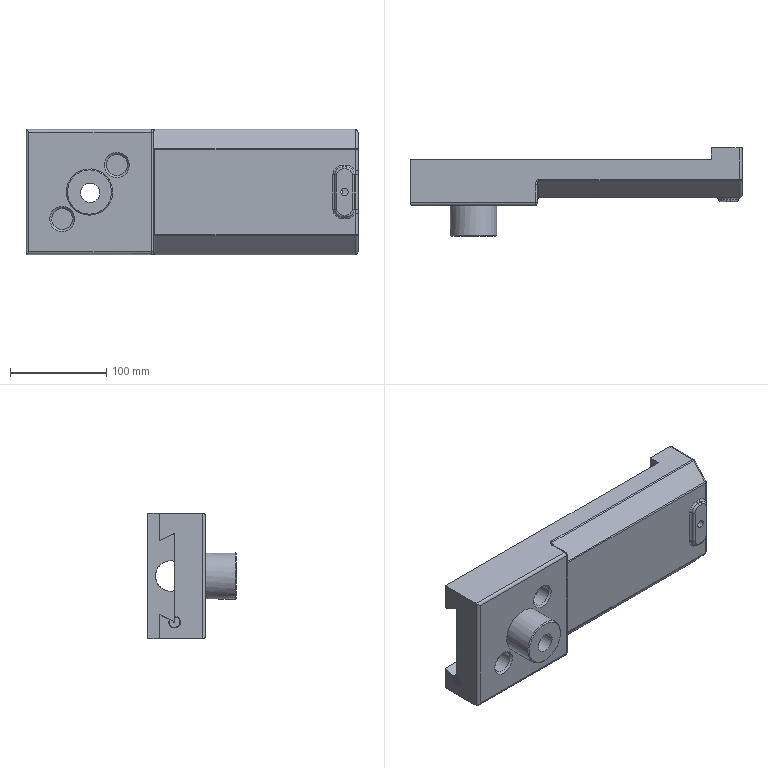Component | NX | TOOL_HOLDER_DOVETAIL_BASE | 1 solid | 175 faces | volume 1158750 mm3 | cylinder 79 | spline 50 | plane 33 | torus 10 | cone 3 | commonest cylinder face diameters 11 x21 12 x20 4 x18 6 x10 8 x4 22 x2 20 x1 48 x1